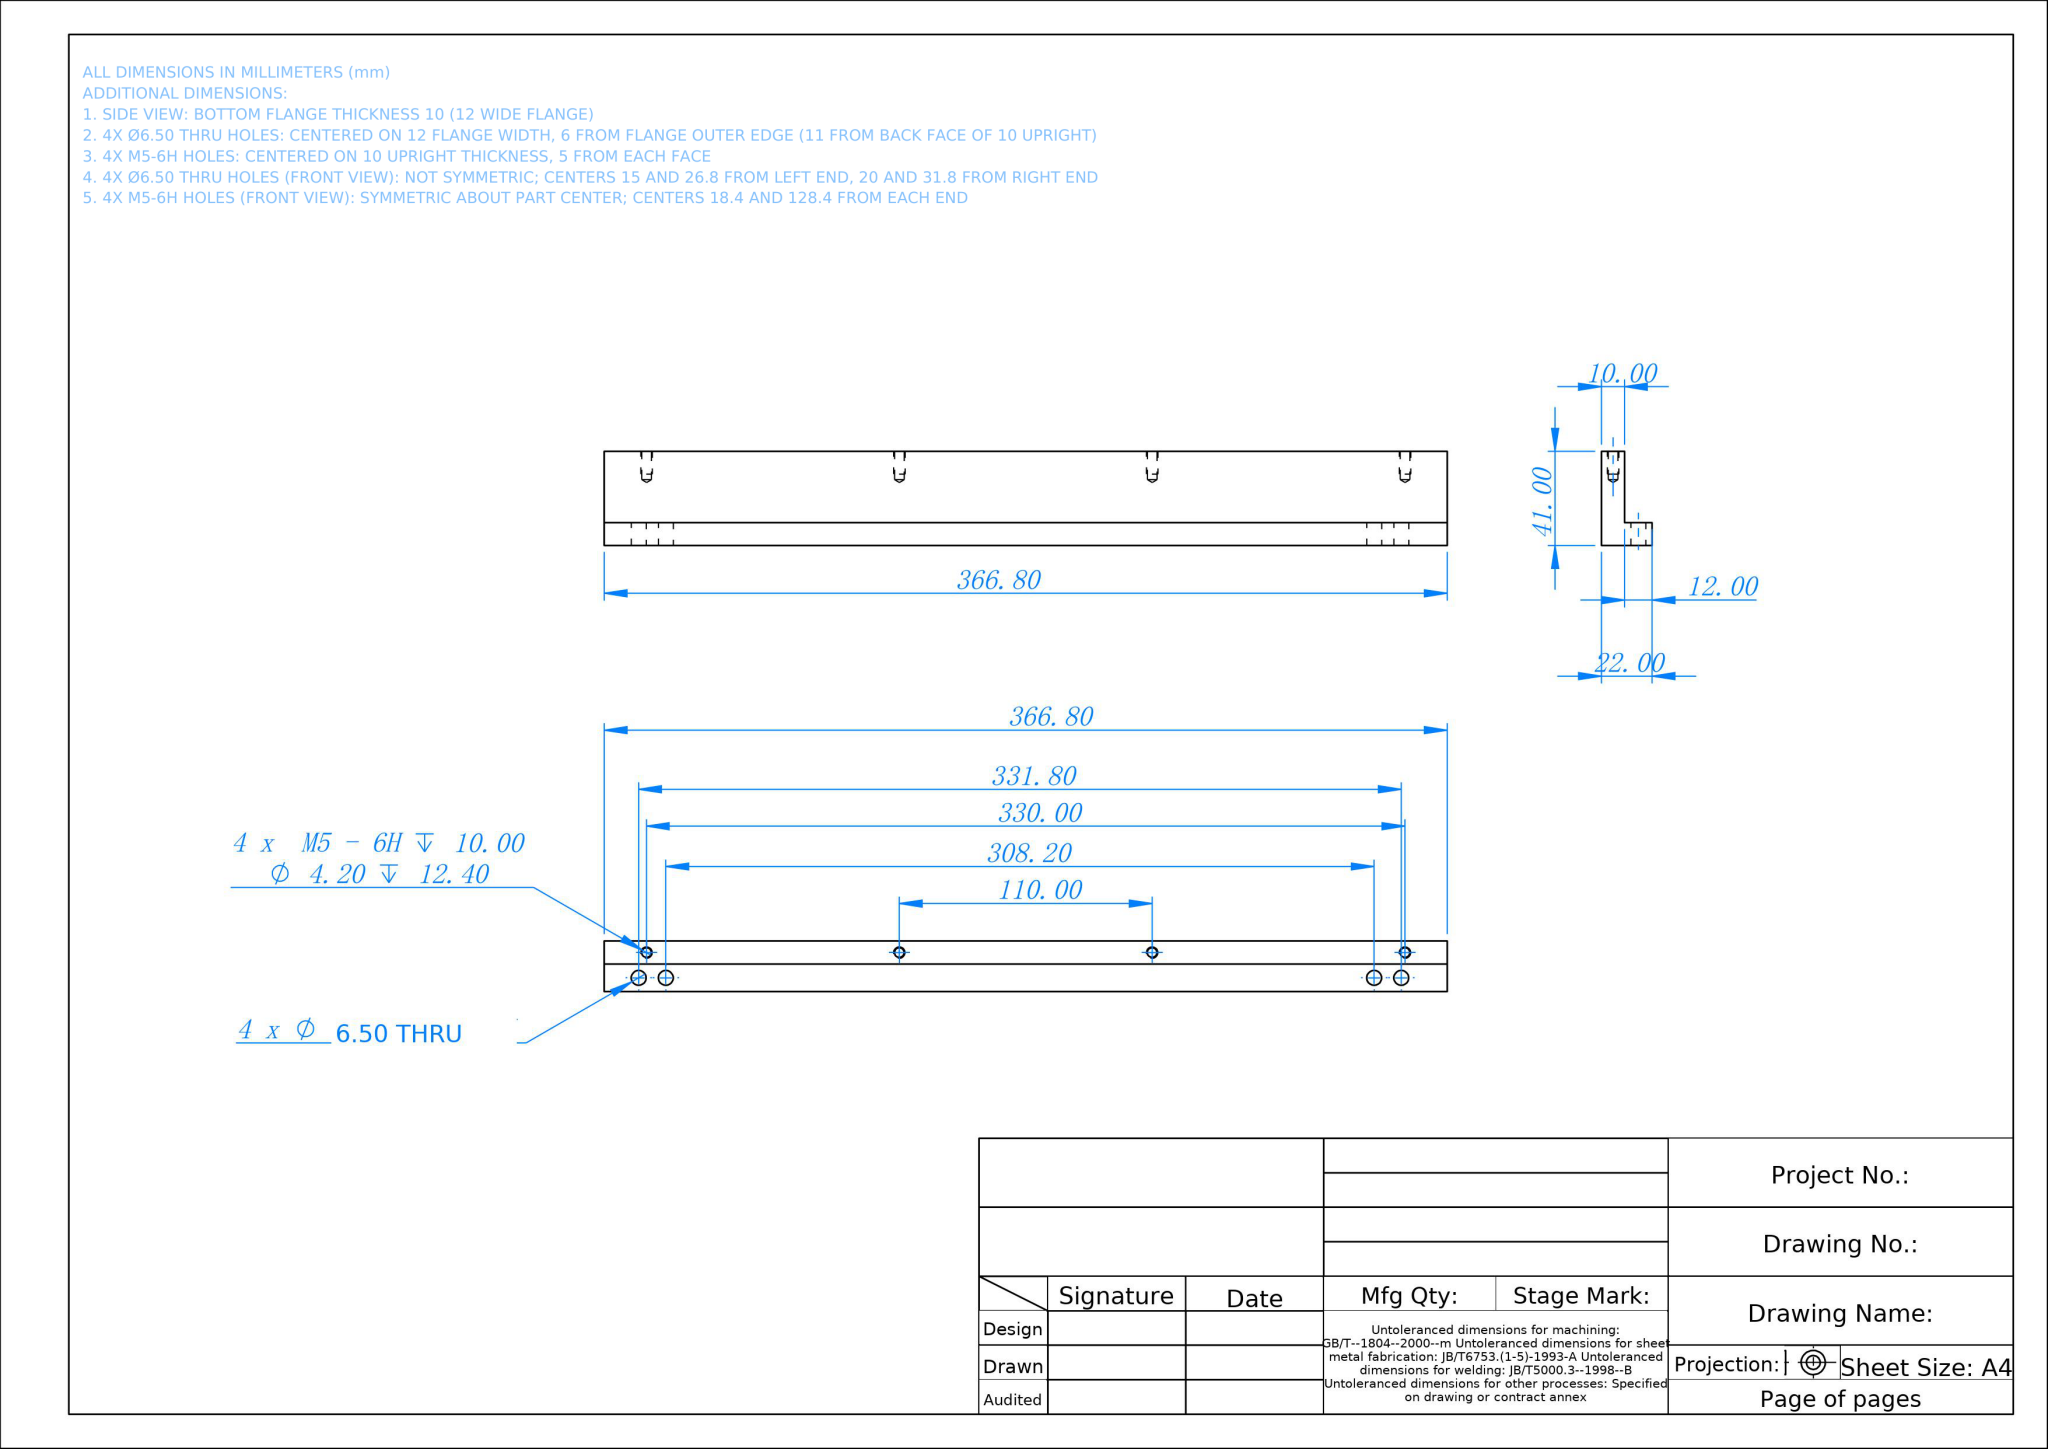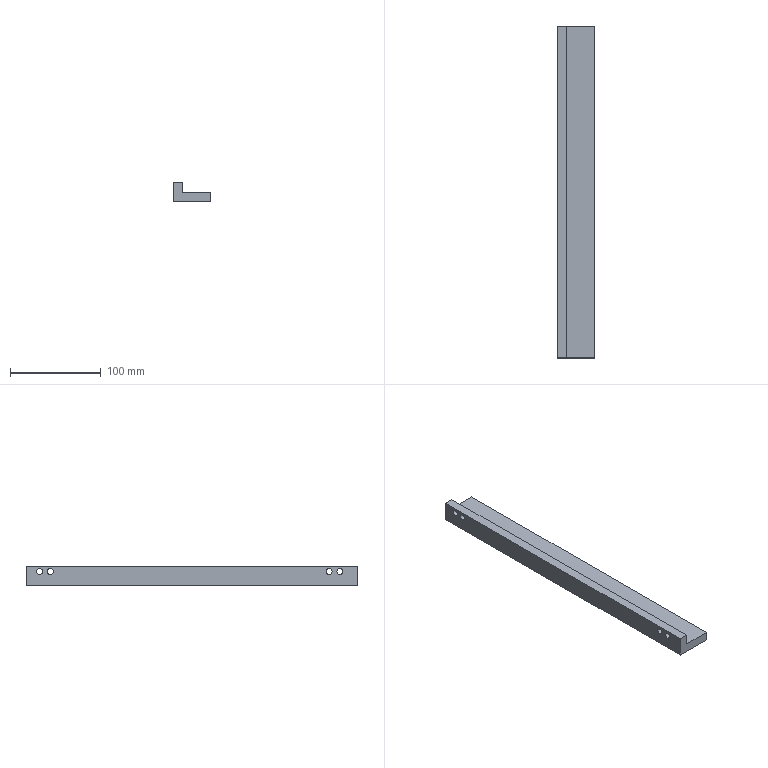Part | NX | mm | 1 solid | 32 faces | box 41 x 366.8 x 22 mm | volume 192366 mm3 | cylinder 16 | cone 8 | plane 8 | commonest cylinder face diameters 6.5 x8 4.2 x8
STEP:
#1=COLOUR_RGB('',0.7922,0.8196,0.9333);
#2=FILL_AREA_STYLE_COLOUR('',#1);
#3=FILL_AREA_STYLE('',(#2));
#4=SURFACE_STYLE_FILL_AREA(#3);
#5=SURFACE_SIDE_STYLE('',(#4));
#6=SURFACE_STYLE_USAGE(.BOTH.,#5);
#7=PRESENTATION_STYLE_ASSIGNMENT((#6));
#8=CARTESIAN_POINT('',(-20.5,168.4,14.25));
#9=VERTEX_POINT('',#8);
#10=CARTESIAN_POINT('',(-20.5,168.4,7.75));
#11=VERTEX_POINT('',#10);
#12=CARTESIAN_POINT('',(-20.5,168.4,11.));
#13=DIRECTION('',(1.,0.,0.));
#14=DIRECTION('',(0.,0.,-1.));
#15=AXIS2_PLACEMENT_3D('',#12,#13,#14);
#16=CIRCLE('',#15,3.25);
#17=EDGE_CURVE('',#9,#11,#16,.T.);
#18=ORIENTED_EDGE('',*,*,#17,.F.);
#19=CARTESIAN_POINT('',(-10.5,168.4,14.25));
#20=VERTEX_POINT('',#19);
#21=CARTESIAN_POINT('',(-10.5,168.4,14.25));
#22=DIRECTION('',(1.,0.,0.));
#23=VECTOR('',#22,1000.);
#24=LINE('',#21,#23);
#25=EDGE_CURVE('',#9,#20,#24,.T.);
#26=ORIENTED_EDGE('',*,*,#25,.T.);
#27=CARTESIAN_POINT('',(-10.5,168.4,7.75));
#28=VERTEX_POINT('',#27);
#29=CARTESIAN_POINT('',(-10.5,168.4,11.));
#30=DIRECTION('',(1.,0.,0.));
#31=DIRECTION('',(0.,0.,-1.));
#32=AXIS2_PLACEMENT_3D('',#29,#30,#31);
#33=CIRCLE('',#32,3.25);
#34=EDGE_CURVE('',#20,#28,#33,.T.);
#35=ORIENTED_EDGE('',*,*,#34,.T.);
#36=CARTESIAN_POINT('',(-10.5,168.4,7.75));
#37=DIRECTION('',(1.,0.,0.));
#38=VECTOR('',#37,1000.);
#39=LINE('',#36,#38);
#40=EDGE_CURVE('',#11,#28,#39,.T.);
#41=ORIENTED_EDGE('',*,*,#40,.F.);
#42=EDGE_LOOP('',(#18,#26,#35,#41));
#43=FACE_OUTER_BOUND('',#42,.T.);
#44=CARTESIAN_POINT('',(-10.5,168.4,11.));
#45=DIRECTION('',(1.,0.,0.));
#46=DIRECTION('',(0.,0.,-1.));
#47=AXIS2_PLACEMENT_3D('',#44,#45,#46);
#48=CYLINDRICAL_SURFACE('',#47,3.25);
#49=ADVANCED_FACE('',(#43),#48,.F.);
#50=CARTESIAN_POINT('',(-20.5,-151.6,14.25));
#51=VERTEX_POINT('',#50);
#52=CARTESIAN_POINT('',(-20.5,-151.6,7.75));
#53=VERTEX_POINT('',#52);
#54=CARTESIAN_POINT('',(-20.5,-151.6,11.));
#55=DIRECTION('',(1.,0.,0.));
#56=DIRECTION('',(0.,0.,-1.));
#57=AXIS2_PLACEMENT_3D('',#54,#55,#56);
#58=CIRCLE('',#57,3.25);
#59=EDGE_CURVE('',#51,#53,#58,.T.);
#60=ORIENTED_EDGE('',*,*,#59,.F.);
#61=CARTESIAN_POINT('',(-10.5,-151.6,14.25));
#62=VERTEX_POINT('',#61);
#63=CARTESIAN_POINT('',(-10.5,-151.6,14.25));
#64=DIRECTION('',(1.,0.,0.));
#65=VECTOR('',#64,1000.);
#66=LINE('',#63,#65);
#67=EDGE_CURVE('',#51,#62,#66,.T.);
#68=ORIENTED_EDGE('',*,*,#67,.T.);
#69=CARTESIAN_POINT('',(-10.5,-151.6,7.75));
#70=VERTEX_POINT('',#69);
#71=CARTESIAN_POINT('',(-10.5,-151.6,11.));
#72=DIRECTION('',(1.,0.,0.));
#73=DIRECTION('',(0.,0.,-1.));
#74=AXIS2_PLACEMENT_3D('',#71,#72,#73);
#75=CIRCLE('',#74,3.25);
#76=EDGE_CURVE('',#62,#70,#75,.T.);
#77=ORIENTED_EDGE('',*,*,#76,.T.);
#78=CARTESIAN_POINT('',(-10.5,-151.6,7.75));
#79=DIRECTION('',(1.,0.,0.));
#80=VECTOR('',#79,1000.);
#81=LINE('',#78,#80);
#82=EDGE_CURVE('',#53,#70,#81,.T.);
#83=ORIENTED_EDGE('',*,*,#82,.F.);
#84=EDGE_LOOP('',(#60,#68,#77,#83));
#85=FACE_OUTER_BOUND('',#84,.T.);
#86=CARTESIAN_POINT('',(-10.5,-151.6,11.));
#87=DIRECTION('',(1.,0.,0.));
#88=DIRECTION('',(0.,0.,-1.));
#89=AXIS2_PLACEMENT_3D('',#86,#87,#88);
#90=CYLINDRICAL_SURFACE('',#89,3.25);
#91=ADVANCED_FACE('',(#85),#90,.F.);
#92=CARTESIAN_POINT('',(-20.5,-163.4,14.25));
#93=VERTEX_POINT('',#92);
#94=CARTESIAN_POINT('',(-20.5,-163.4,7.75));
#95=VERTEX_POINT('',#94);
#96=CARTESIAN_POINT('',(-20.5,-163.4,11.));
#97=DIRECTION('',(1.,0.,0.));
#98=DIRECTION('',(0.,0.,-1.));
#99=AXIS2_PLACEMENT_3D('',#96,#97,#98);
#100=CIRCLE('',#99,3.25);
#101=EDGE_CURVE('',#93,#95,#100,.T.);
#102=ORIENTED_EDGE('',*,*,#101,.F.);
#103=CARTESIAN_POINT('',(-10.5,-163.4,14.25));
#104=VERTEX_POINT('',#103);
#105=CARTESIAN_POINT('',(-10.5,-163.4,14.25));
#106=DIRECTION('',(1.,0.,0.));
#107=VECTOR('',#106,1000.);
#108=LINE('',#105,#107);
#109=EDGE_CURVE('',#93,#104,#108,.T.);
#110=ORIENTED_EDGE('',*,*,#109,.T.);
#111=CARTESIAN_POINT('',(-10.5,-163.4,7.75));
#112=VERTEX_POINT('',#111);
#113=CARTESIAN_POINT('',(-10.5,-163.4,11.));
#114=DIRECTION('',(1.,0.,0.));
#115=DIRECTION('',(0.,0.,-1.));
#116=AXIS2_PLACEMENT_3D('',#113,#114,#115);
#117=CIRCLE('',#116,3.25);
#118=EDGE_CURVE('',#104,#112,#117,.T.);
#119=ORIENTED_EDGE('',*,*,#118,.T.);
#120=CARTESIAN_POINT('',(-10.5,-163.4,7.75));
#121=DIRECTION('',(1.,0.,0.));
#122=VECTOR('',#121,1000.);
#123=LINE('',#120,#122);
#124=EDGE_CURVE('',#95,#112,#123,.T.);
#125=ORIENTED_EDGE('',*,*,#124,.F.);
#126=EDGE_LOOP('',(#102,#110,#119,#125));
#127=FACE_OUTER_BOUND('',#126,.T.);
#128=CARTESIAN_POINT('',(-10.5,-163.4,11.));
#129=DIRECTION('',(1.,0.,0.));
#130=DIRECTION('',(0.,0.,-1.));
#131=AXIS2_PLACEMENT_3D('',#128,#129,#130);
#132=CYLINDRICAL_SURFACE('',#131,3.25);
#133=ADVANCED_FACE('',(#127),#132,.F.);
#134=CARTESIAN_POINT('',(-20.5,156.6,14.25));
#135=VERTEX_POINT('',#134);
#136=CARTESIAN_POINT('',(-20.5,156.6,7.75));
#137=VERTEX_POINT('',#136);
#138=CARTESIAN_POINT('',(-20.5,156.6,11.));
#139=DIRECTION('',(1.,0.,0.));
#140=DIRECTION('',(0.,0.,-1.));
#141=AXIS2_PLACEMENT_3D('',#138,#139,#140);
#142=CIRCLE('',#141,3.25);
#143=EDGE_CURVE('',#135,#137,#142,.T.);
#144=ORIENTED_EDGE('',*,*,#143,.F.);
#145=CARTESIAN_POINT('',(-10.5,156.6,14.25));
#146=VERTEX_POINT('',#145);
#147=CARTESIAN_POINT('',(-10.5,156.6,14.25));
#148=DIRECTION('',(1.,0.,0.));
#149=VECTOR('',#148,1000.);
#150=LINE('',#147,#149);
#151=EDGE_CURVE('',#135,#146,#150,.T.);
#152=ORIENTED_EDGE('',*,*,#151,.T.);
#153=CARTESIAN_POINT('',(-10.5,156.6,7.75));
#154=VERTEX_POINT('',#153);
#155=CARTESIAN_POINT('',(-10.5,156.6,11.));
#156=DIRECTION('',(1.,0.,0.));
#157=DIRECTION('',(0.,0.,-1.));
#158=AXIS2_PLACEMENT_3D('',#155,#156,#157);
#159=CIRCLE('',#158,3.25);
#160=EDGE_CURVE('',#146,#154,#159,.T.);
#161=ORIENTED_EDGE('',*,*,#160,.T.);
#162=CARTESIAN_POINT('',(-10.5,156.6,7.75));
#163=DIRECTION('',(1.,0.,0.));
#164=VECTOR('',#163,1000.);
#165=LINE('',#162,#164);
#166=EDGE_CURVE('',#137,#154,#165,.T.);
#167=ORIENTED_EDGE('',*,*,#166,.F.);
#168=EDGE_LOOP('',(#144,#152,#161,#167));
#169=FACE_OUTER_BOUND('',#168,.T.);
#170=CARTESIAN_POINT('',(-10.5,156.6,11.));
#171=DIRECTION('',(1.,0.,0.));
#172=DIRECTION('',(0.,0.,-1.));
#173=AXIS2_PLACEMENT_3D('',#170,#171,#172);
#174=CYLINDRICAL_SURFACE('',#173,3.25);
#175=ADVANCED_FACE('',(#169),#174,.F.);
#176=CARTESIAN_POINT('',(8.1,-165.,2.1));
#177=VERTEX_POINT('',#176);
#178=CARTESIAN_POINT('',(8.1,-165.,-2.1));
#179=VERTEX_POINT('',#178);
#180=CARTESIAN_POINT('',(8.1,-165.,0.));
#181=DIRECTION('',(1.,0.,0.));
#182=DIRECTION('',(0.,0.,-1.));
#183=AXIS2_PLACEMENT_3D('',#180,#181,#182);
#184=CIRCLE('',#183,2.1);
#185=EDGE_CURVE('',#177,#179,#184,.T.);
#186=ORIENTED_EDGE('',*,*,#185,.F.);
#187=CARTESIAN_POINT('',(20.5,-165.,2.1));
#188=VERTEX_POINT('',#187);
#189=CARTESIAN_POINT('',(20.5,-165.,2.1));
#190=DIRECTION('',(1.,0.,0.));
#191=VECTOR('',#190,1000.);
#192=LINE('',#189,#191);
#193=EDGE_CURVE('',#177,#188,#192,.T.);
#194=ORIENTED_EDGE('',*,*,#193,.T.);
#195=CARTESIAN_POINT('',(20.5,-165.,-2.1));
#196=VERTEX_POINT('',#195);
#197=CARTESIAN_POINT('',(20.5,-165.,0.));
#198=DIRECTION('',(1.,0.,0.));
#199=DIRECTION('',(0.,0.,-1.));
#200=AXIS2_PLACEMENT_3D('',#197,#198,#199);
#201=CIRCLE('',#200,2.1);
#202=EDGE_CURVE('',#188,#196,#201,.T.);
#203=ORIENTED_EDGE('',*,*,#202,.T.);
#204=CARTESIAN_POINT('',(20.5,-165.,-2.1));
#205=DIRECTION('',(1.,0.,0.));
#206=VECTOR('',#205,1000.);
#207=LINE('',#204,#206);
#208=EDGE_CURVE('',#179,#196,#207,.T.);
#209=ORIENTED_EDGE('',*,*,#208,.F.);
#210=EDGE_LOOP('',(#186,#194,#203,#209));
#211=FACE_OUTER_BOUND('',#210,.T.);
#212=CARTESIAN_POINT('',(20.5,-165.,0.));
#213=DIRECTION('',(1.,0.,0.));
#214=DIRECTION('',(0.,0.,-1.));
#215=AXIS2_PLACEMENT_3D('',#212,#213,#214);
#216=CYLINDRICAL_SURFACE('',#215,2.1);
#217=ADVANCED_FACE('',(#211),#216,.F.);
#218=CARTESIAN_POINT('',(6.838,-165.,0.));
#219=VERTEX_POINT('',#218);
#220=CARTESIAN_POINT('',(8.1,-165.,-2.1));
#221=DIRECTION('',(0.515,0.,-0.8572));
#222=VECTOR('',#221,1000.);
#223=LINE('',#220,#222);
#224=EDGE_CURVE('',#219,#179,#223,.T.);
#225=ORIENTED_EDGE('',*,*,#224,.F.);
#226=CARTESIAN_POINT('',(8.1,-165.,2.1));
#227=DIRECTION('',(0.515,0.,0.8572));
#228=VECTOR('',#227,1000.);
#229=LINE('',#226,#228);
#230=EDGE_CURVE('',#219,#177,#229,.T.);
#231=ORIENTED_EDGE('',*,*,#230,.T.);
#232=ORIENTED_EDGE('',*,*,#185,.T.);
#233=EDGE_LOOP('',(#225,#231,#232));
#234=FACE_OUTER_BOUND('',#233,.T.);
#235=CARTESIAN_POINT('',(8.1,-165.,0.));
#236=DIRECTION('',(1.,0.,0.));
#237=DIRECTION('',(0.,0.,-1.));
#238=AXIS2_PLACEMENT_3D('',#235,#236,#237);
#239=CONICAL_SURFACE('',#238,2.1,1.03);
#240=ADVANCED_FACE('',(#234),#239,.F.);
#241=CARTESIAN_POINT('',(8.1,-55.,2.1));
#242=VERTEX_POINT('',#241);
#243=CARTESIAN_POINT('',(8.1,-55.,-2.1));
#244=VERTEX_POINT('',#243);
#245=CARTESIAN_POINT('',(8.1,-55.,-0.));
#246=DIRECTION('',(1.,0.,0.));
#247=DIRECTION('',(0.,0.,-1.));
#248=AXIS2_PLACEMENT_3D('',#245,#246,#247);
#249=CIRCLE('',#248,2.1);
#250=EDGE_CURVE('',#242,#244,#249,.T.);
#251=ORIENTED_EDGE('',*,*,#250,.F.);
#252=CARTESIAN_POINT('',(20.5,-55.,2.1));
#253=VERTEX_POINT('',#252);
#254=CARTESIAN_POINT('',(20.5,-55.,2.1));
#255=DIRECTION('',(1.,0.,0.));
#256=VECTOR('',#255,1000.);
#257=LINE('',#254,#256);
#258=EDGE_CURVE('',#242,#253,#257,.T.);
#259=ORIENTED_EDGE('',*,*,#258,.T.);
#260=CARTESIAN_POINT('',(20.5,-55.,-2.1));
#261=VERTEX_POINT('',#260);
#262=CARTESIAN_POINT('',(20.5,-55.,-0.));
#263=DIRECTION('',(1.,0.,0.));
#264=DIRECTION('',(0.,0.,-1.));
#265=AXIS2_PLACEMENT_3D('',#262,#263,#264);
#266=CIRCLE('',#265,2.1);
#267=EDGE_CURVE('',#253,#261,#266,.T.);
#268=ORIENTED_EDGE('',*,*,#267,.T.);
#269=CARTESIAN_POINT('',(20.5,-55.,-2.1));
#270=DIRECTION('',(1.,0.,0.));
#271=VECTOR('',#270,1000.);
#272=LINE('',#269,#271);
#273=EDGE_CURVE('',#244,#261,#272,.T.);
#274=ORIENTED_EDGE('',*,*,#273,.F.);
#275=EDGE_LOOP('',(#251,#259,#268,#274));
#276=FACE_OUTER_BOUND('',#275,.T.);
#277=CARTESIAN_POINT('',(20.5,-55.,-0.));
#278=DIRECTION('',(1.,0.,0.));
#279=DIRECTION('',(0.,0.,-1.));
#280=AXIS2_PLACEMENT_3D('',#277,#278,#279);
#281=CYLINDRICAL_SURFACE('',#280,2.1);
#282=ADVANCED_FACE('',(#276),#281,.F.);
#283=CARTESIAN_POINT('',(6.838,-55.,-0.));
#284=VERTEX_POINT('',#283);
#285=CARTESIAN_POINT('',(8.1,-55.,-2.1));
#286=DIRECTION('',(0.515,0.,-0.8572));
#287=VECTOR('',#286,1000.);
#288=LINE('',#285,#287);
#289=EDGE_CURVE('',#284,#244,#288,.T.);
#290=ORIENTED_EDGE('',*,*,#289,.F.);
#291=CARTESIAN_POINT('',(8.1,-55.,2.1));
#292=DIRECTION('',(0.515,0.,0.8572));
#293=VECTOR('',#292,1000.);
#294=LINE('',#291,#293);
#295=EDGE_CURVE('',#284,#242,#294,.T.);
#296=ORIENTED_EDGE('',*,*,#295,.T.);
#297=ORIENTED_EDGE('',*,*,#250,.T.);
#298=EDGE_LOOP('',(#290,#296,#297));
#299=FACE_OUTER_BOUND('',#298,.T.);
#300=CARTESIAN_POINT('',(8.1,-55.,-0.));
#301=DIRECTION('',(1.,0.,0.));
#302=DIRECTION('',(0.,0.,-1.));
#303=AXIS2_PLACEMENT_3D('',#300,#301,#302);
#304=CONICAL_SURFACE('',#303,2.1,1.03);
#305=ADVANCED_FACE('',(#299),#304,.F.);
#306=CARTESIAN_POINT('',(8.1,165.,2.1));
#307=VERTEX_POINT('',#306);
#308=CARTESIAN_POINT('',(8.1,165.,-2.1));
#309=VERTEX_POINT('',#308);
#310=CARTESIAN_POINT('',(8.1,165.,0.));
#311=DIRECTION('',(1.,0.,0.));
#312=DIRECTION('',(0.,0.,-1.));
#313=AXIS2_PLACEMENT_3D('',#310,#311,#312);
#314=CIRCLE('',#313,2.1);
#315=EDGE_CURVE('',#307,#309,#314,.T.);
#316=ORIENTED_EDGE('',*,*,#315,.F.);
#317=CARTESIAN_POINT('',(20.5,165.,2.1));
#318=VERTEX_POINT('',#317);
#319=CARTESIAN_POINT('',(20.5,165.,2.1));
#320=DIRECTION('',(1.,0.,0.));
#321=VECTOR('',#320,1000.);
#322=LINE('',#319,#321);
#323=EDGE_CURVE('',#307,#318,#322,.T.);
#324=ORIENTED_EDGE('',*,*,#323,.T.);
#325=CARTESIAN_POINT('',(20.5,165.,-2.1));
#326=VERTEX_POINT('',#325);
#327=CARTESIAN_POINT('',(20.5,165.,0.));
#328=DIRECTION('',(1.,0.,0.));
#329=DIRECTION('',(0.,0.,-1.));
#330=AXIS2_PLACEMENT_3D('',#327,#328,#329);
#331=CIRCLE('',#330,2.1);
#332=EDGE_CURVE('',#318,#326,#331,.T.);
#333=ORIENTED_EDGE('',*,*,#332,.T.);
#334=CARTESIAN_POINT('',(20.5,165.,-2.1));
#335=DIRECTION('',(1.,0.,0.));
#336=VECTOR('',#335,1000.);
#337=LINE('',#334,#336);
#338=EDGE_CURVE('',#309,#326,#337,.T.);
#339=ORIENTED_EDGE('',*,*,#338,.F.);
#340=EDGE_LOOP('',(#316,#324,#333,#339));
#341=FACE_OUTER_BOUND('',#340,.T.);
#342=CARTESIAN_POINT('',(20.5,165.,0.));
#343=DIRECTION('',(1.,0.,0.));
#344=DIRECTION('',(0.,0.,-1.));
#345=AXIS2_PLACEMENT_3D('',#342,#343,#344);
#346=CYLINDRICAL_SURFACE('',#345,2.1);
#347=ADVANCED_FACE('',(#341),#346,.F.);
#348=CARTESIAN_POINT('',(6.838,165.,0.));
#349=VERTEX_POINT('',#348);
#350=CARTESIAN_POINT('',(8.1,165.,-2.1));
#351=DIRECTION('',(0.515,0.,-0.8572));
#352=VECTOR('',#351,1000.);
#353=LINE('',#350,#352);
#354=EDGE_CURVE('',#349,#309,#353,.T.);
#355=ORIENTED_EDGE('',*,*,#354,.F.);
#356=CARTESIAN_POINT('',(8.1,165.,2.1));
#357=DIRECTION('',(0.515,0.,0.8572));
#358=VECTOR('',#357,1000.);
#359=LINE('',#356,#358);
#360=EDGE_CURVE('',#349,#307,#359,.T.);
#361=ORIENTED_EDGE('',*,*,#360,.T.);
#362=ORIENTED_EDGE('',*,*,#315,.T.);
#363=EDGE_LOOP('',(#355,#361,#362));
#364=FACE_OUTER_BOUND('',#363,.T.);
#365=CARTESIAN_POINT('',(8.1,165.,0.));
#366=DIRECTION('',(1.,0.,0.));
#367=DIRECTION('',(0.,0.,-1.));
#368=AXIS2_PLACEMENT_3D('',#365,#366,#367);
#369=CONICAL_SURFACE('',#368,2.1,1.03);
#370=ADVANCED_FACE('',(#364),#369,.F.);
#371=CARTESIAN_POINT('',(8.1,55.,2.1));
#372=VERTEX_POINT('',#371);
#373=CARTESIAN_POINT('',(8.1,55.,-2.1));
#374=VERTEX_POINT('',#373);
#375=CARTESIAN_POINT('',(8.1,55.,0.));
#376=DIRECTION('',(1.,0.,0.));
#377=DIRECTION('',(0.,0.,-1.));
#378=AXIS2_PLACEMENT_3D('',#375,#376,#377);
#379=CIRCLE('',#378,2.1);
#380=EDGE_CURVE('',#372,#374,#379,.T.);
#381=ORIENTED_EDGE('',*,*,#380,.F.);
#382=CARTESIAN_POINT('',(20.5,55.,2.1));
#383=VERTEX_POINT('',#382);
#384=CARTESIAN_POINT('',(20.5,55.,2.1));
#385=DIRECTION('',(1.,0.,0.));
#386=VECTOR('',#385,1000.);
#387=LINE('',#384,#386);
#388=EDGE_CURVE('',#372,#383,#387,.T.);
#389=ORIENTED_EDGE('',*,*,#388,.T.);
#390=CARTESIAN_POINT('',(20.5,55.,-2.1));
#391=VERTEX_POINT('',#390);
#392=CARTESIAN_POINT('',(20.5,55.,0.));
#393=DIRECTION('',(1.,0.,0.));
#394=DIRECTION('',(0.,0.,-1.));
#395=AXIS2_PLACEMENT_3D('',#392,#393,#394);
#396=CIRCLE('',#395,2.1);
#397=EDGE_CURVE('',#383,#391,#396,.T.);
#398=ORIENTED_EDGE('',*,*,#397,.T.);
#399=CARTESIAN_POINT('',(20.5,55.,-2.1));
#400=DIRECTION('',(1.,0.,0.));
#401=VECTOR('',#400,1000.);
#402=LINE('',#399,#401);
#403=EDGE_CURVE('',#374,#391,#402,.T.);
#404=ORIENTED_EDGE('',*,*,#403,.F.);
#405=EDGE_LOOP('',(#381,#389,#398,#404));
#406=FACE_OUTER_BOUND('',#405,.T.);
#407=CARTESIAN_POINT('',(20.5,55.,0.));
#408=DIRECTION('',(1.,0.,0.));
#409=DIRECTION('',(0.,0.,-1.));
#410=AXIS2_PLACEMENT_3D('',#407,#408,#409);
#411=CYLINDRICAL_SURFACE('',#410,2.1);
#412=ADVANCED_FACE('',(#406),#411,.F.);
#413=CARTESIAN_POINT('',(6.838,55.,0.));
#414=VERTEX_POINT('',#413);
#415=CARTESIAN_POINT('',(8.1,55.,-2.1));
#416=DIRECTION('',(0.515,0.,-0.8572));
#417=VECTOR('',#416,1000.);
#418=LINE('',#415,#417);
#419=EDGE_CURVE('',#414,#374,#418,.T.);
#420=ORIENTED_EDGE('',*,*,#419,.F.);
#421=CARTESIAN_POINT('',(8.1,55.,2.1));
#422=DIRECTION('',(0.515,0.,0.8572));
#423=VECTOR('',#422,1000.);
#424=LINE('',#421,#423);
#425=EDGE_CURVE('',#414,#372,#424,.T.);
#426=ORIENTED_EDGE('',*,*,#425,.T.);
#427=ORIENTED_EDGE('',*,*,#380,.T.);
#428=EDGE_LOOP('',(#420,#426,#427));
#429=FACE_OUTER_BOUND('',#428,.T.);
#430=CARTESIAN_POINT('',(8.1,55.,0.));
#431=DIRECTION('',(1.,0.,0.));
#432=DIRECTION('',(0.,0.,-1.));
#433=AXIS2_PLACEMENT_3D('',#430,#431,#432);
#434=CONICAL_SURFACE('',#433,2.1,1.03);
#435=ADVANCED_FACE('',(#429),#434,.F.);
#436=CARTESIAN_POINT('',(-10.5,-183.4,5.));
#437=VERTEX_POINT('',#436);
#438=CARTESIAN_POINT('',(-10.5,183.4,5.));
#439=VERTEX_POINT('',#438);
#440=CARTESIAN_POINT('',(-10.5,183.4,5.));
#441=DIRECTION('',(-0.,1.,0.));
#442=VECTOR('',#441,1000.);
#443=LINE('',#440,#442);
#444=EDGE_CURVE('',#437,#439,#443,.T.);
#445=ORIENTED_EDGE('',*,*,#444,.F.);
#446=CARTESIAN_POINT('',(20.5,-183.4,5.));
#447=VERTEX_POINT('',#446);
#448=CARTESIAN_POINT('',(-20.5,-183.4,5.));
#449=DIRECTION('',(1.,0.,0.));
#450=VECTOR('',#449,1000.);
#451=LINE('',#448,#450);
#452=EDGE_CURVE('',#437,#447,#451,.T.);
#453=ORIENTED_EDGE('',*,*,#452,.T.);
#454=CARTESIAN_POINT('',(20.5,183.4,5.));
#455=VERTEX_POINT('',#454);
#456=CARTESIAN_POINT('',(20.5,-183.4,5.));
#457=DIRECTION('',(0.,1.,0.));
#458=VECTOR('',#457,1000.);
#459=LINE('',#456,#458);
#460=EDGE_CURVE('',#447,#455,#459,.T.);
#461=ORIENTED_EDGE('',*,*,#460,.T.);
#462=CARTESIAN_POINT('',(-20.5,183.4,5.));
#463=DIRECTION('',(-1.,0.,0.));
#464=VECTOR('',#463,1000.);
#465=LINE('',#462,#464);
#466=EDGE_CURVE('',#455,#439,#465,.T.);
#467=ORIENTED_EDGE('',*,*,#466,.T.);
#468=EDGE_LOOP('',(#445,#453,#461,#467));
#469=FACE_OUTER_BOUND('',#468,.T.);
#470=CARTESIAN_POINT('',(0.,0.,5.));
#471=DIRECTION('',(0.,0.,-1.));
#472=DIRECTION('',(-1.,0.,0.));
#473=AXIS2_PLACEMENT_3D('',#470,#471,#472);
#474=PLANE('',#473);
#475=ADVANCED_FACE('',(#469),#474,.F.);
#476=CARTESIAN_POINT('',(20.5,-165.,0.));
#477=DIRECTION('',(1.,0.,0.));
#478=DIRECTION('',(0.,0.,-1.));
#479=AXIS2_PLACEMENT_3D('',#476,#477,#478);
#480=CIRCLE('',#479,2.1);
#481=EDGE_CURVE('',#196,#188,#480,.T.);
#482=ORIENTED_EDGE('',*,*,#481,.F.);
#483=ORIENTED_EDGE('',*,*,#202,.F.);
#484=EDGE_LOOP('',(#482,#483));
#485=FACE_BOUND('',#484,.T.);
#486=CARTESIAN_POINT('',(20.5,-55.,-0.));
#487=DIRECTION('',(1.,0.,0.));
#488=DIRECTION('',(0.,0.,-1.));
#489=AXIS2_PLACEMENT_3D('',#486,#487,#488);
#490=CIRCLE('',#489,2.1);
#491=EDGE_CURVE('',#261,#253,#490,.T.);
#492=ORIENTED_EDGE('',*,*,#491,.F.);
#493=ORIENTED_EDGE('',*,*,#267,.F.);
#494=EDGE_LOOP('',(#492,#493));
#495=FACE_BOUND('',#494,.T.);
#496=CARTESIAN_POINT('',(20.5,165.,0.));
#497=DIRECTION('',(1.,0.,0.));
#498=DIRECTION('',(0.,0.,-1.));
#499=AXIS2_PLACEMENT_3D('',#496,#497,#498);
#500=CIRCLE('',#499,2.1);
#501=EDGE_CURVE('',#326,#318,#500,.T.);
#502=ORIENTED_EDGE('',*,*,#501,.F.);
#503=ORIENTED_EDGE('',*,*,#332,.F.);
#504=EDGE_LOOP('',(#502,#503));
#505=FACE_BOUND('',#504,.T.);
#506=CARTESIAN_POINT('',(20.5,55.,0.));
#507=DIRECTION('',(1.,0.,0.));
#508=DIRECTION('',(0.,0.,-1.));
#509=AXIS2_PLACEMENT_3D('',#506,#507,#508);
#510=CIRCLE('',#509,2.1);
#511=EDGE_CURVE('',#391,#383,#510,.T.);
#512=ORIENTED_EDGE('',*,*,#511,.F.);
#513=ORIENTED_EDGE('',*,*,#397,.F.);
#514=EDGE_LOOP('',(#512,#513));
#515=FACE_BOUND('',#514,.T.);
#516=CARTESIAN_POINT('',(20.5,-183.4,-5.));
#517=VERTEX_POINT('',#516);
#518=CARTESIAN_POINT('',(20.5,183.4,-5.));
#519=VERTEX_POINT('',#518);
#520=CARTESIAN_POINT('',(20.5,-183.4,-5.));
#521=DIRECTION('',(0.,1.,0.));
#522=VECTOR('',#521,1000.);
#523=LINE('',#520,#522);
#524=EDGE_CURVE('',#517,#519,#523,.T.);
#525=ORIENTED_EDGE('',*,*,#524,.T.);
#526=CARTESIAN_POINT('',(20.5,183.4,5.));
#527=DIRECTION('',(0.,0.,-1.));
#528=VECTOR('',#527,1000.);
#529=LINE('',#526,#528);
#530=EDGE_CURVE('',#455,#519,#529,.T.);
#531=ORIENTED_EDGE('',*,*,#530,.F.);
#532=ORIENTED_EDGE('',*,*,#460,.F.);
#533=CARTESIAN_POINT('',(20.5,-183.4,5.));
#534=DIRECTION('',(0.,0.,-1.));
#535=VECTOR('',#534,1000.);
#536=LINE('',#533,#535);
#537=EDGE_CURVE('',#447,#517,#536,.T.);
#538=ORIENTED_EDGE('',*,*,#537,.T.);
#539=EDGE_LOOP('',(#525,#531,#532,#538));
#540=FACE_OUTER_BOUND('',#539,.T.);
#541=CARTESIAN_POINT('',(20.5,-183.4,5.));
#542=DIRECTION('',(-1.,0.,0.));
#543=DIRECTION('',(0.,0.,1.));
#544=AXIS2_PLACEMENT_3D('',#541,#542,#543);
#545=PLANE('',#544);
#546=ADVANCED_FACE('',(#485,#495,#505,#515,#540),#545,.F.);
#547=CARTESIAN_POINT('',(-20.5,183.4,-5.));
#548=VERTEX_POINT('',#547);
#549=CARTESIAN_POINT('',(-20.5,183.4,-5.));
#550=DIRECTION('',(-1.,0.,0.));
#551=VECTOR('',#550,1000.);
#552=LINE('',#549,#551);
#553=EDGE_CURVE('',#519,#548,#552,.T.);
#554=ORIENTED_EDGE('',*,*,#553,.T.);
#555=CARTESIAN_POINT('',(-20.5,183.4,17.));
#556=VERTEX_POINT('',#555);
#557=CARTESIAN_POINT('',(-20.5,183.4,5.));
#558=DIRECTION('',(0.,0.,-1.));
#559=VECTOR('',#558,1000.);
#560=LINE('',#557,#559);
#561=EDGE_CURVE('',#556,#548,#560,.T.);
#562=ORIENTED_EDGE('',*,*,#561,.F.);
#563=CARTESIAN_POINT('',(-10.5,183.4,17.));
#564=VERTEX_POINT('',#563);
#565=CARTESIAN_POINT('',(-20.5,183.4,17.));
#566=DIRECTION('',(-1.,0.,0.));
#567=VECTOR('',#566,1000.);
#568=LINE('',#565,#567);
#569=EDGE_CURVE('',#564,#556,#568,.T.);
#570=ORIENTED_EDGE('',*,*,#569,.F.);
#571=CARTESIAN_POINT('',(-10.5,183.4,17.));
#572=DIRECTION('',(0.,0.,-1.));
#573=VECTOR('',#572,1000.);
#574=LINE('',#571,#573);
#575=EDGE_CURVE('',#564,#439,#574,.T.);
#576=ORIENTED_EDGE('',*,*,#575,.T.);
#577=ORIENTED_EDGE('',*,*,#466,.F.);
#578=ORIENTED_EDGE('',*,*,#530,.T.);
#579=EDGE_LOOP('',(#554,#562,#570,#576,#577,#578));
#580=FACE_OUTER_BOUND('',#579,.T.);
#581=CARTESIAN_POINT('',(-20.5,183.4,5.));
#582=DIRECTION('',(0.,-1.,0.));
#583=DIRECTION('',(0.,0.,-1.));
#584=AXIS2_PLACEMENT_3D('',#581,#582,#583);
#585=PLANE('',#584);
#586=ADVANCED_FACE('',(#580),#585,.F.);
#587=CARTESIAN_POINT('',(-20.5,168.4,11.));
#588=DIRECTION('',(1.,0.,0.));
#589=DIRECTION('',(0.,0.,-1.));
#590=AXIS2_PLACEMENT_3D('',#587,#588,#589);
#591=CIRCLE('',#590,3.25);
#592=EDGE_CURVE('',#11,#9,#591,.T.);
#593=ORIENTED_EDGE('',*,*,#592,.T.);
#594=ORIENTED_EDGE('',*,*,#17,.T.);
#595=EDGE_LOOP('',(#593,#594));
#596=FACE_BOUND('',#595,.T.);
#597=CARTESIAN_POINT('',(-20.5,-151.6,11.));
#598=DIRECTION('',(1.,0.,0.));
#599=DIRECTION('',(0.,0.,-1.));
#600=AXIS2_PLACEMENT_3D('',#597,#598,#599);
#601=CIRCLE('',#600,3.25);
#602=EDGE_CURVE('',#53,#51,#601,.T.);
#603=ORIENTED_EDGE('',*,*,#602,.T.);
#604=ORIENTED_EDGE('',*,*,#59,.T.);
#605=EDGE_LOOP('',(#603,#604));
#606=FACE_BOUND('',#605,.T.);
#607=CARTESIAN_POINT('',(-20.5,-163.4,11.));
#608=DIRECTION('',(1.,0.,0.));
#609=DIRECTION('',(0.,0.,-1.));
#610=AXIS2_PLACEMENT_3D('',#607,#608,#609);
#611=CIRCLE('',#610,3.25);
#612=EDGE_CURVE('',#95,#93,#611,.T.);
#613=ORIENTED_EDGE('',*,*,#612,.T.);
#614=ORIENTED_EDGE('',*,*,#101,.T.);
#615=EDGE_LOOP('',(#613,#614));
#616=FACE_BOUND('',#615,.T.);
#617=CARTESIAN_POINT('',(-20.5,156.6,11.));
#618=DIRECTION('',(1.,0.,0.));
#619=DIRECTION('',(0.,0.,-1.));
#620=AXIS2_PLACEMENT_3D('',#617,#618,#619);
#621=CIRCLE('',#620,3.25);
#622=EDGE_CURVE('',#137,#135,#621,.T.);
#623=ORIENTED_EDGE('',*,*,#622,.T.);
#624=ORIENTED_EDGE('',*,*,#143,.T.);
#625=EDGE_LOOP('',(#623,#624));
#626=FACE_BOUND('',#625,.T.);
#627=CARTESIAN_POINT('',(-20.5,-183.4,-5.));
#628=VERTEX_POINT('',#627);
#629=CARTESIAN_POINT('',(-20.5,-183.4,-5.));
#630=DIRECTION('',(0.,-1.,0.));
#631=VECTOR('',#630,1000.);
#632=LINE('',#629,#631);
#633=EDGE_CURVE('',#548,#628,#632,.T.);
#634=ORIENTED_EDGE('',*,*,#633,.T.);
#635=CARTESIAN_POINT('',(-20.5,-183.4,17.));
#636=VERTEX_POINT('',#635);
#637=CARTESIAN_POINT('',(-20.5,-183.4,5.));
#638=DIRECTION('',(0.,0.,-1.));
#639=VECTOR('',#638,1000.);
#640=LINE('',#637,#639);
#641=EDGE_CURVE('',#636,#628,#640,.T.);
#642=ORIENTED_EDGE('',*,*,#641,.F.);
#643=CARTESIAN_POINT('',(-20.5,183.4,17.));
#644=DIRECTION('',(0.,-1.,0.));
#645=VECTOR('',#644,1000.);
#646=LINE('',#643,#645);
#647=EDGE_CURVE('',#556,#636,#646,.T.);
#648=ORIENTED_EDGE('',*,*,#647,.F.);
#649=ORIENTED_EDGE('',*,*,#561,.T.);
#650=EDGE_LOOP('',(#634,#642,#648,#649));
#651=FACE_OUTER_BOUND('',#650,.T.);
#652=CARTESIAN_POINT('',(-20.5,-183.4,5.));
#653=DIRECTION('',(1.,0.,0.));
#654=DIRECTION('',(0.,0.,-1.));
#655=AXIS2_PLACEMENT_3D('',#652,#653,#654);
#656=PLANE('',#655);
#657=ADVANCED_FACE('',(#596,#606,#616,#626,#651),#656,.F.);
#658=CARTESIAN_POINT('',(-20.5,-183.4,-5.));
#659=DIRECTION('',(1.,0.,0.));
#660=VECTOR('',#659,1000.);
#661=LINE('',#658,#660);
#662=EDGE_CURVE('',#628,#517,#661,.T.);
#663=ORIENTED_EDGE('',*,*,#662,.T.);
#664=ORIENTED_EDGE('',*,*,#537,.F.);
#665=ORIENTED_EDGE('',*,*,#452,.F.);
#666=CARTESIAN_POINT('',(-10.5,-183.4,17.));
#667=VERTEX_POINT('',#666);
#668=CARTESIAN_POINT('',(-10.5,-183.4,17.));
#669=DIRECTION('',(0.,0.,-1.));
#670=VECTOR('',#669,1000.);
#671=LINE('',#668,#670);
#672=EDGE_CURVE('',#667,#437,#671,.T.);
#673=ORIENTED_EDGE('',*,*,#672,.F.);
#674=CARTESIAN_POINT('',(-20.5,-183.4,17.));
#675=DIRECTION('',(1.,0.,0.));
#676=VECTOR('',#675,1000.);
#677=LINE('',#674,#676);
#678=EDGE_CURVE('',#636,#667,#677,.T.);
#679=ORIENTED_EDGE('',*,*,#678,.F.);
#680=ORIENTED_EDGE('',*,*,#641,.T.);
#681=EDGE_LOOP('',(#663,#664,#665,#673,#679,#680));
#682=FACE_OUTER_BOUND('',#681,.T.);
#683=CARTESIAN_POINT('',(-20.5,-183.4,5.));
#684=DIRECTION('',(0.,1.,0.));
#685=DIRECTION('',(0.,0.,1.));
#686=AXIS2_PLACEMENT_3D('',#683,#684,#685);
#687=PLANE('',#686);
#688=ADVANCED_FACE('',(#682),#687,.F.);
#689=ORIENTED_EDGE('',*,*,#524,.F.);
#690=ORIENTED_EDGE('',*,*,#662,.F.);
#691=ORIENTED_EDGE('',*,*,#633,.F.);
#692=ORIENTED_EDGE('',*,*,#553,.F.);
#693=EDGE_LOOP('',(#689,#690,#691,#692));
#694=FACE_OUTER_BOUND('',#693,.T.);
#695=CARTESIAN_POINT('',(0.,0.,-5.));
#696=DIRECTION('',(0.,0.,-1.));
#697=DIRECTION('',(-1.,0.,0.));
#698=AXIS2_PLACEMENT_3D('',#695,#696,#697);
#699=PLANE('',#698);
#700=ADVANCED_FACE('',(#694),#699,.T.);
#701=CARTESIAN_POINT('',(-10.5,168.4,11.));
#702=DIRECTION('',(1.,0.,0.));
#703=DIRECTION('',(0.,0.,-1.));
#704=AXIS2_PLACEMENT_3D('',#701,#702,#703);
#705=CIRCLE('',#704,3.25);
#706=EDGE_CURVE('',#28,#20,#705,.T.);
#707=ORIENTED_EDGE('',*,*,#706,.F.);
#708=ORIENTED_EDGE('',*,*,#34,.F.);
#709=EDGE_LOOP('',(#707,#708));
#710=FACE_BOUND('',#709,.T.);
#711=CARTESIAN_POINT('',(-10.5,-151.6,11.));
#712=DIRECTION('',(1.,0.,0.));
#713=DIRECTION('',(0.,0.,-1.));
#714=AXIS2_PLACEMENT_3D('',#711,#712,#713);
#715=CIRCLE('',#714,3.25);
#716=EDGE_CURVE('',#70,#62,#715,.T.);
#717=ORIENTED_EDGE('',*,*,#716,.F.);
#718=ORIENTED_EDGE('',*,*,#76,.F.);
#719=EDGE_LOOP('',(#717,#718));
#720=FACE_BOUND('',#719,.T.);
#721=CARTESIAN_POINT('',(-10.5,-163.4,11.));
#722=DIRECTION('',(1.,0.,0.));
#723=DIRECTION('',(0.,0.,-1.));
#724=AXIS2_PLACEMENT_3D('',#721,#722,#723);
#725=CIRCLE('',#724,3.25);
#726=EDGE_CURVE('',#112,#104,#725,.T.);
#727=ORIENTED_EDGE('',*,*,#726,.F.);
#728=ORIENTED_EDGE('',*,*,#118,.F.);
#729=EDGE_LOOP('',(#727,#728));
#730=FACE_BOUND('',#729,.T.);
#731=CARTESIAN_POINT('',(-10.5,156.6,11.));
#732=DIRECTION('',(1.,0.,0.));
#733=DIRECTION('',(0.,0.,-1.));
#734=AXIS2_PLACEMENT_3D('',#731,#732,#733);
#735=CIRCLE('',#734,3.25);
#736=EDGE_CURVE('',#154,#146,#735,.T.);
#737=ORIENTED_EDGE('',*,*,#736,.F.);
#738=ORIENTED_EDGE('',*,*,#160,.F.);
#739=EDGE_LOOP('',(#737,#738));
#740=FACE_BOUND('',#739,.T.);
#741=ORIENTED_EDGE('',*,*,#444,.T.);
#742=ORIENTED_EDGE('',*,*,#575,.F.);
#743=CARTESIAN_POINT('',(-10.5,183.4,17.));
#744=DIRECTION('',(-0.,1.,0.));
#745=VECTOR('',#744,1000.);
#746=LINE('',#743,#745);
#747=EDGE_CURVE('',#667,#564,#746,.T.);
#748=ORIENTED_EDGE('',*,*,#747,.F.);
#749=ORIENTED_EDGE('',*,*,#672,.T.);
#750=EDGE_LOOP('',(#741,#742,#748,#749));
#751=FACE_OUTER_BOUND('',#750,.T.);
#752=CARTESIAN_POINT('',(-10.5,183.4,17.));
#753=DIRECTION('',(-1.,-0.,0.));
#754=DIRECTION('',(0.,-1.,0.));
#755=AXIS2_PLACEMENT_3D('',#752,#753,#754);
#756=PLANE('',#755);
#757=ADVANCED_FACE('',(#710,#720,#730,#740,#751),#756,.F.);
#758=ORIENTED_EDGE('',*,*,#647,.T.);
#759=ORIENTED_EDGE('',*,*,#678,.T.);
#760=ORIENTED_EDGE('',*,*,#747,.T.);
#761=ORIENTED_EDGE('',*,*,#569,.T.);
#762=EDGE_LOOP('',(#758,#759,#760,#761));
#763=FACE_OUTER_BOUND('',#762,.T.);
#764=CARTESIAN_POINT('',(0.,0.,17.));
#765=DIRECTION('',(0.,0.,1.));
#766=DIRECTION('',(1.,0.,0.));
#767=AXIS2_PLACEMENT_3D('',#764,#765,#766);
#768=PLANE('',#767);
#769=ADVANCED_FACE('',(#763),#768,.T.);
#770=ORIENTED_EDGE('',*,*,#425,.F.);
#771=ORIENTED_EDGE('',*,*,#419,.T.);
#772=CARTESIAN_POINT('',(8.1,55.,0.));
#773=DIRECTION('',(1.,0.,0.));
#774=DIRECTION('',(0.,0.,-1.));
#775=AXIS2_PLACEMENT_3D('',#772,#773,#774);
#776=CIRCLE('',#775,2.1);
#777=EDGE_CURVE('',#374,#372,#776,.T.);
#778=ORIENTED_EDGE('',*,*,#777,.T.);
#779=EDGE_LOOP('',(#770,#771,#778));
#780=FACE_OUTER_BOUND('',#779,.T.);
#781=CARTESIAN_POINT('',(8.1,55.,0.));
#782=DIRECTION('',(1.,0.,0.));
#783=DIRECTION('',(0.,0.,-1.));
#784=AXIS2_PLACEMENT_3D('',#781,#782,#783);
#785=CONICAL_SURFACE('',#784,2.1,1.03);
#786=ADVANCED_FACE('',(#780),#785,.F.);
#787=ORIENTED_EDGE('',*,*,#388,.F.);
#788=ORIENTED_EDGE('',*,*,#777,.F.);
#789=ORIENTED_EDGE('',*,*,#403,.T.);
#790=ORIENTED_EDGE('',*,*,#511,.T.);
#791=EDGE_LOOP('',(#787,#788,#789,#790));
#792=FACE_OUTER_BOUND('',#791,.T.);
#793=CARTESIAN_POINT('',(20.5,55.,0.));
#794=DIRECTION('',(1.,0.,0.));
#795=DIRECTION('',(0.,0.,-1.));
#796=AXIS2_PLACEMENT_3D('',#793,#794,#795);
#797=CYLINDRICAL_SURFACE('',#796,2.1);
#798=ADVANCED_FACE('',(#792),#797,.F.);
#799=ORIENTED_EDGE('',*,*,#360,.F.);
#800=ORIENTED_EDGE('',*,*,#354,.T.);
#801=CARTESIAN_POINT('',(8.1,165.,0.));
#802=DIRECTION('',(1.,0.,0.));
#803=DIRECTION('',(0.,0.,-1.));
#804=AXIS2_PLACEMENT_3D('',#801,#802,#803);
#805=CIRCLE('',#804,2.1);
#806=EDGE_CURVE('',#309,#307,#805,.T.);
#807=ORIENTED_EDGE('',*,*,#806,.T.);
#808=EDGE_LOOP('',(#799,#800,#807));
#809=FACE_OUTER_BOUND('',#808,.T.);
#810=CARTESIAN_POINT('',(8.1,165.,0.));
#811=DIRECTION('',(1.,0.,0.));
#812=DIRECTION('',(0.,0.,-1.));
#813=AXIS2_PLACEMENT_3D('',#810,#811,#812);
#814=CONICAL_SURFACE('',#813,2.1,1.03);
#815=ADVANCED_FACE('',(#809),#814,.F.);
#816=ORIENTED_EDGE('',*,*,#323,.F.);
#817=ORIENTED_EDGE('',*,*,#806,.F.);
#818=ORIENTED_EDGE('',*,*,#338,.T.);
#819=ORIENTED_EDGE('',*,*,#501,.T.);
#820=EDGE_LOOP('',(#816,#817,#818,#819));
#821=FACE_OUTER_BOUND('',#820,.T.);
#822=CARTESIAN_POINT('',(20.5,165.,0.));
#823=DIRECTION('',(1.,0.,0.));
#824=DIRECTION('',(0.,0.,-1.));
#825=AXIS2_PLACEMENT_3D('',#822,#823,#824);
#826=CYLINDRICAL_SURFACE('',#825,2.1);
#827=ADVANCED_FACE('',(#821),#826,.F.);
#828=ORIENTED_EDGE('',*,*,#295,.F.);
#829=ORIENTED_EDGE('',*,*,#289,.T.);
#830=CARTESIAN_POINT('',(8.1,-55.,-0.));
#831=DIRECTION('',(1.,0.,0.));
#832=DIRECTION('',(0.,0.,-1.));
#833=AXIS2_PLACEMENT_3D('',#830,#831,#832);
#834=CIRCLE('',#833,2.1);
#835=EDGE_CURVE('',#244,#242,#834,.T.);
#836=ORIENTED_EDGE('',*,*,#835,.T.);
#837=EDGE_LOOP('',(#828,#829,#836));
#838=FACE_OUTER_BOUND('',#837,.T.);
#839=CARTESIAN_POINT('',(8.1,-55.,-0.));
#840=DIRECTION('',(1.,0.,0.));
#841=DIRECTION('',(0.,0.,-1.));
#842=AXIS2_PLACEMENT_3D('',#839,#840,#841);
#843=CONICAL_SURFACE('',#842,2.1,1.03);
#844=ADVANCED_FACE('',(#838),#843,.F.);
#845=ORIENTED_EDGE('',*,*,#258,.F.);
#846=ORIENTED_EDGE('',*,*,#835,.F.);
#847=ORIENTED_EDGE('',*,*,#273,.T.);
#848=ORIENTED_EDGE('',*,*,#491,.T.);
#849=EDGE_LOOP('',(#845,#846,#847,#848));
#850=FACE_OUTER_BOUND('',#849,.T.);
#851=CARTESIAN_POINT('',(20.5,-55.,-0.));
#852=DIRECTION('',(1.,0.,0.));
#853=DIRECTION('',(0.,0.,-1.));
#854=AXIS2_PLACEMENT_3D('',#851,#852,#853);
#855=CYLINDRICAL_SURFACE('',#854,2.1);
#856=ADVANCED_FACE('',(#850),#855,.F.);
#857=ORIENTED_EDGE('',*,*,#230,.F.);
#858=ORIENTED_EDGE('',*,*,#224,.T.);
#859=CARTESIAN_POINT('',(8.1,-165.,0.));
#860=DIRECTION('',(1.,0.,0.));
#861=DIRECTION('',(0.,0.,-1.));
#862=AXIS2_PLACEMENT_3D('',#859,#860,#861);
#863=CIRCLE('',#862,2.1);
#864=EDGE_CURVE('',#179,#177,#863,.T.);
#865=ORIENTED_EDGE('',*,*,#864,.T.);
#866=EDGE_LOOP('',(#857,#858,#865));
#867=FACE_OUTER_BOUND('',#866,.T.);
#868=CARTESIAN_POINT('',(8.1,-165.,0.));
#869=DIRECTION('',(1.,0.,0.));
#870=DIRECTION('',(0.,0.,-1.));
#871=AXIS2_PLACEMENT_3D('',#868,#869,#870);
#872=CONICAL_SURFACE('',#871,2.1,1.03);
#873=ADVANCED_FACE('',(#867),#872,.F.);
#874=ORIENTED_EDGE('',*,*,#193,.F.);
#875=ORIENTED_EDGE('',*,*,#864,.F.);
#876=ORIENTED_EDGE('',*,*,#208,.T.);
#877=ORIENTED_EDGE('',*,*,#481,.T.);
#878=EDGE_LOOP('',(#874,#875,#876,#877));
#879=FACE_OUTER_BOUND('',#878,.T.);
#880=CARTESIAN_POINT('',(20.5,-165.,0.));
#881=DIRECTION('',(1.,0.,0.));
#882=DIRECTION('',(0.,0.,-1.));
#883=AXIS2_PLACEMENT_3D('',#880,#881,#882);
#884=CYLINDRICAL_SURFACE('',#883,2.1);
#885=ADVANCED_FACE('',(#879),#884,.F.);
#886=ORIENTED_EDGE('',*,*,#151,.F.);
#887=ORIENTED_EDGE('',*,*,#622,.F.);
#888=ORIENTED_EDGE('',*,*,#166,.T.);
#889=ORIENTED_EDGE('',*,*,#736,.T.);
#890=EDGE_LOOP('',(#886,#887,#888,#889));
#891=FACE_OUTER_BOUND('',#890,.T.);
#892=CARTESIAN_POINT('',(-10.5,156.6,11.));
#893=DIRECTION('',(1.,0.,0.));
#894=DIRECTION('',(0.,0.,-1.));
#895=AXIS2_PLACEMENT_3D('',#892,#893,#894);
#896=CYLINDRICAL_SURFACE('',#895,3.25);
#897=ADVANCED_FACE('',(#891),#896,.F.);
#898=ORIENTED_EDGE('',*,*,#109,.F.);
#899=ORIENTED_EDGE('',*,*,#612,.F.);
#900=ORIENTED_EDGE('',*,*,#124,.T.);
#901=ORIENTED_EDGE('',*,*,#726,.T.);
#902=EDGE_LOOP('',(#898,#899,#900,#901));
#903=FACE_OUTER_BOUND('',#902,.T.);
#904=CARTESIAN_POINT('',(-10.5,-163.4,11.));
#905=DIRECTION('',(1.,0.,0.));
#906=DIRECTION('',(0.,0.,-1.));
#907=AXIS2_PLACEMENT_3D('',#904,#905,#906);
#908=CYLINDRICAL_SURFACE('',#907,3.25);
#909=ADVANCED_FACE('',(#903),#908,.F.);
#910=ORIENTED_EDGE('',*,*,#67,.F.);
#911=ORIENTED_EDGE('',*,*,#602,.F.);
#912=ORIENTED_EDGE('',*,*,#82,.T.);
#913=ORIENTED_EDGE('',*,*,#716,.T.);
#914=EDGE_LOOP('',(#910,#911,#912,#913));
#915=FACE_OUTER_BOUND('',#914,.T.);
#916=CARTESIAN_POINT('',(-10.5,-151.6,11.));
#917=DIRECTION('',(1.,0.,0.));
#918=DIRECTION('',(0.,0.,-1.));
#919=AXIS2_PLACEMENT_3D('',#916,#917,#918);
#920=CYLINDRICAL_SURFACE('',#919,3.25);
#921=ADVANCED_FACE('',(#915),#920,.F.);
#922=ORIENTED_EDGE('',*,*,#25,.F.);
#923=ORIENTED_EDGE('',*,*,#592,.F.);
#924=ORIENTED_EDGE('',*,*,#40,.T.);
#925=ORIENTED_EDGE('',*,*,#706,.T.);
#926=EDGE_LOOP('',(#922,#923,#924,#925));
#927=FACE_OUTER_BOUND('',#926,.T.);
#928=CARTESIAN_POINT('',(-10.5,168.4,11.));
#929=DIRECTION('',(1.,0.,0.));
#930=DIRECTION('',(0.,0.,-1.));
#931=AXIS2_PLACEMENT_3D('',#928,#929,#930);
#932=CYLINDRICAL_SURFACE('',#931,3.25);
#933=ADVANCED_FACE('',(#927),#932,.F.);
#934=CLOSED_SHELL('',(#49,#91,#133,#175,#217,#240,#282,#305,#347,#370,#412,#435,#475,#546,#586,#657,#688,#700,#757,#769,#786,#798,#815,#827,#844,#856,#873,#885,#897,#909,#921,#933));
#935=MANIFOLD_SOLID_BREP('',#934);
#936=STYLED_ITEM('',(#7),#935);
#937=PRESENTATION_LAYER_ASSIGNMENT('','',(#936));
#938=CARTESIAN_POINT('',(0.,0.,0.));
#939=DIRECTION('',(0.,0.,1.));
#940=DIRECTION('',(1.,0.,0.));
#941=AXIS2_PLACEMENT_3D('',#938,#939,#940);
#942=(LENGTH_UNIT()NAMED_UNIT(*)SI_UNIT(.MILLI.,.METRE.));
#943=UNCERTAINTY_MEASURE_WITH_UNIT(LENGTH_MEASURE(0.00001),#942,'','');
#944=(NAMED_UNIT(*)PLANE_ANGLE_UNIT()SI_UNIT($,.RADIAN.));
#945=(NAMED_UNIT(*)SI_UNIT($,.STERADIAN.)SOLID_ANGLE_UNIT());
#946=(GEOMETRIC_REPRESENTATION_CONTEXT(3)GLOBAL_UNCERTAINTY_ASSIGNED_CONTEXT((#943))GLOBAL_UNIT_ASSIGNED_CONTEXT((#942,#944,#945))REPRESENTATION_CONTEXT('',''));
#947=ADVANCED_BREP_SHAPE_REPRESENTATION('',(#935,#941),#946);
#948=(LENGTH_UNIT()NAMED_UNIT(*)SI_UNIT(.MILLI.,.METRE.));
#949=UNCERTAINTY_MEASURE_WITH_UNIT(LENGTH_MEASURE(0.00001),#948,'','');
#950=(NAMED_UNIT(*)PLANE_ANGLE_UNIT()SI_UNIT($,.RADIAN.));
#951=(NAMED_UNIT(*)SI_UNIT($,.STERADIAN.)SOLID_ANGLE_UNIT());
#952=(GEOMETRIC_REPRESENTATION_CONTEXT(3)GLOBAL_UNCERTAINTY_ASSIGNED_CONTEXT((#949))GLOBAL_UNIT_ASSIGNED_CONTEXT((#948,#950,#951))REPRESENTATION_CONTEXT('',''));
#953=MECHANICAL_DESIGN_GEOMETRIC_PRESENTATION_REPRESENTATION('',(#936),#952);